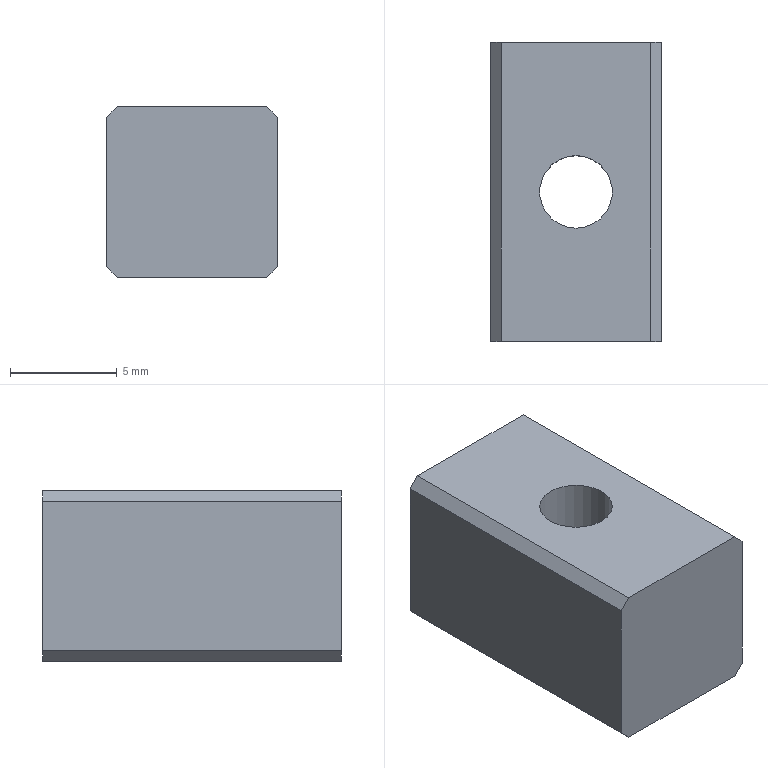Component | NX | LOCATING_KEY | 1 solid | 13 faces | box 8 x 14 x 8 mm | volume 732 mm3 | plane 11 | cylinder 2 | commonest cylinder face diameters 3.4 x1 6.5 x1
STEP:
#1=CARTESIAN_POINT('',(0.,0.,0.));
#2=DIRECTION('',(0.,0.,1.));
#3=DIRECTION('',(1.,0.,0.));
#4=AXIS2_PLACEMENT_3D('',#1,#2,#3);
#5=CARTESIAN_POINT('',(-3.5,90.,-0.));
#6=VERTEX_POINT('',#5);
#7=CARTESIAN_POINT('',(3.5,90.,-0.));
#8=VERTEX_POINT('',#7);
#9=CARTESIAN_POINT('',(-4.,90.,-0.));
#10=DIRECTION('',(1.,0.,0.));
#11=VECTOR('',#10,1.);
#12=LINE('',#9,#11);
#13=CARTESIAN_POINT('',(-4.,90.,-0.));
#14=DIRECTION('',(0.,1.,0.));
#15=DIRECTION('',(0.,0.,-1.));
#16=AXIS2_PLACEMENT_3D('',#13,#14,#15);
#17=PLANE('',#16);
#18=CARTESIAN_POINT('',(0.,0.));
#19=DIRECTION('',(0.,-1.));
#20=VECTOR('',#19,1.);
#21=LINE('',#18,#20);
#22=(GEOMETRIC_REPRESENTATION_CONTEXT(2)PARAMETRIC_REPRESENTATION_CONTEXT()REPRESENTATION_CONTEXT('',''));
#23=DEFINITIONAL_REPRESENTATION('',(#21),#22);
#24=PCURVE('',#17,#23);
#25=CARTESIAN_POINT('',(0.,97.,-0.));
#26=DIRECTION('',(0.,0.,1.));
#27=DIRECTION('',(0.,1.,0.));
#28=AXIS2_PLACEMENT_3D('',#25,#26,#27);
#29=PLANE('',#28);
#30=CARTESIAN_POINT('',(-7.,4.));
#31=DIRECTION('',(0.,-1.));
#32=VECTOR('',#31,1.);
#33=LINE('',#30,#32);
#34=(GEOMETRIC_REPRESENTATION_CONTEXT(2)PARAMETRIC_REPRESENTATION_CONTEXT()REPRESENTATION_CONTEXT('',''));
#35=DEFINITIONAL_REPRESENTATION('',(#33),#34);
#36=PCURVE('',#29,#35);
#37=SURFACE_CURVE('',#12,(#24,#36),.PCURVE_S1.);
#38=EDGE_CURVE('',#6,#8,#37,.T.);
#39=ORIENTED_EDGE('',*,*,#38,.F.);
#40=CARTESIAN_POINT('',(-4.,90.,-0.5));
#41=VERTEX_POINT('',#40);
#42=CARTESIAN_POINT('',(-3.5,90.,-0.));
#43=DIRECTION('',(-0.7071,0.,-0.7071));
#44=VECTOR('',#43,1.);
#45=LINE('',#42,#44);
#46=CARTESIAN_POINT('',(0.,-0.5));
#47=DIRECTION('',(0.7071,0.7071));
#48=VECTOR('',#47,1.);
#49=LINE('',#46,#48);
#50=(GEOMETRIC_REPRESENTATION_CONTEXT(2)PARAMETRIC_REPRESENTATION_CONTEXT()REPRESENTATION_CONTEXT('',''));
#51=DEFINITIONAL_REPRESENTATION('',(#49),#50);
#52=PCURVE('',#17,#51);
#53=CARTESIAN_POINT('',(-3.5,97.,-0.));
#54=DIRECTION('',(-0.7071,0.,0.7071));
#55=DIRECTION('',(0.,1.,0.));
#56=AXIS2_PLACEMENT_3D('',#53,#54,#55);
#57=PLANE('',#56);
#58=CARTESIAN_POINT('',(-7.,0.));
#59=DIRECTION('',(0.,1.));
#60=VECTOR('',#59,1.);
#61=LINE('',#58,#60);
#62=(GEOMETRIC_REPRESENTATION_CONTEXT(2)PARAMETRIC_REPRESENTATION_CONTEXT()REPRESENTATION_CONTEXT('',''));
#63=DEFINITIONAL_REPRESENTATION('',(#61),#62);
#64=PCURVE('',#57,#63);
#65=SURFACE_CURVE('',#45,(#52,#64),.PCURVE_S1.);
#66=EDGE_CURVE('',#6,#41,#65,.T.);
#67=ORIENTED_EDGE('',*,*,#66,.T.);
#68=CARTESIAN_POINT('',(-4.,90.,-7.5));
#69=VERTEX_POINT('',#68);
#70=CARTESIAN_POINT('',(-4.,90.,-0.));
#71=DIRECTION('',(0.,0.,-1.));
#72=VECTOR('',#71,1.);
#73=LINE('',#70,#72);
#74=CARTESIAN_POINT('',(0.,0.));
#75=DIRECTION('',(1.,0.));
#76=VECTOR('',#75,1.);
#77=LINE('',#74,#76);
#78=(GEOMETRIC_REPRESENTATION_CONTEXT(2)PARAMETRIC_REPRESENTATION_CONTEXT()REPRESENTATION_CONTEXT('',''));
#79=DEFINITIONAL_REPRESENTATION('',(#77),#78);
#80=PCURVE('',#17,#79);
#81=CARTESIAN_POINT('',(-4.,104.,-0.));
#82=DIRECTION('',(1.,0.,0.));
#83=DIRECTION('',(0.,0.,-1.));
#84=AXIS2_PLACEMENT_3D('',#81,#82,#83);
#85=PLANE('',#84);
#86=CARTESIAN_POINT('',(0.,-14.));
#87=DIRECTION('',(1.,0.));
#88=VECTOR('',#87,1.);
#89=LINE('',#86,#88);
#90=(GEOMETRIC_REPRESENTATION_CONTEXT(2)PARAMETRIC_REPRESENTATION_CONTEXT()REPRESENTATION_CONTEXT('',''));
#91=DEFINITIONAL_REPRESENTATION('',(#89),#90);
#92=PCURVE('',#85,#91);
#93=SURFACE_CURVE('',#73,(#80,#92),.PCURVE_S1.);
#94=EDGE_CURVE('',#41,#69,#93,.T.);
#95=ORIENTED_EDGE('',*,*,#94,.T.);
#96=CARTESIAN_POINT('',(-3.5,90.,-8.));
#97=VERTEX_POINT('',#96);
#98=CARTESIAN_POINT('',(-4.,90.,-7.5));
#99=DIRECTION('',(0.7071,0.,-0.7071));
#100=VECTOR('',#99,1.);
#101=LINE('',#98,#100);
#102=CARTESIAN_POINT('',(7.5,0.));
#103=DIRECTION('',(0.7071,-0.7071));
#104=VECTOR('',#103,1.);
#105=LINE('',#102,#104);
#106=(GEOMETRIC_REPRESENTATION_CONTEXT(2)PARAMETRIC_REPRESENTATION_CONTEXT()REPRESENTATION_CONTEXT('',''));
#107=DEFINITIONAL_REPRESENTATION('',(#105),#106);
#108=PCURVE('',#17,#107);
#109=CARTESIAN_POINT('',(-4.,104.,-7.5));
#110=DIRECTION('',(0.7071,0.,0.7071));
#111=DIRECTION('',(0.,-1.,0.));
#112=AXIS2_PLACEMENT_3D('',#109,#110,#111);
#113=PLANE('',#112);
#114=CARTESIAN_POINT('',(14.,0.));
#115=DIRECTION('',(0.,1.));
#116=VECTOR('',#115,1.);
#117=LINE('',#114,#116);
#118=(GEOMETRIC_REPRESENTATION_CONTEXT(2)PARAMETRIC_REPRESENTATION_CONTEXT()REPRESENTATION_CONTEXT('',''));
#119=DEFINITIONAL_REPRESENTATION('',(#117),#118);
#120=PCURVE('',#113,#119);
#121=SURFACE_CURVE('',#101,(#108,#120),.PCURVE_S1.);
#122=EDGE_CURVE('',#69,#97,#121,.T.);
#123=ORIENTED_EDGE('',*,*,#122,.T.);
#124=CARTESIAN_POINT('',(3.5,90.,-8.));
#125=VERTEX_POINT('',#124);
#126=CARTESIAN_POINT('',(-4.,90.,-8.));
#127=DIRECTION('',(1.,0.,0.));
#128=VECTOR('',#127,1.);
#129=LINE('',#126,#128);
#130=CARTESIAN_POINT('',(8.,0.));
#131=DIRECTION('',(0.,-1.));
#132=VECTOR('',#131,1.);
#133=LINE('',#130,#132);
#134=(GEOMETRIC_REPRESENTATION_CONTEXT(2)PARAMETRIC_REPRESENTATION_CONTEXT()REPRESENTATION_CONTEXT('',''));
#135=DEFINITIONAL_REPRESENTATION('',(#133),#134);
#136=PCURVE('',#17,#135);
#137=CARTESIAN_POINT('',(0.,97.,-8.));
#138=DIRECTION('',(0.,0.,1.));
#139=DIRECTION('',(0.,1.,0.));
#140=AXIS2_PLACEMENT_3D('',#137,#138,#139);
#141=PLANE('',#140);
#142=CARTESIAN_POINT('',(-7.,4.));
#143=DIRECTION('',(0.,-1.));
#144=VECTOR('',#143,1.);
#145=LINE('',#142,#144);
#146=(GEOMETRIC_REPRESENTATION_CONTEXT(2)PARAMETRIC_REPRESENTATION_CONTEXT()REPRESENTATION_CONTEXT('',''));
#147=DEFINITIONAL_REPRESENTATION('',(#145),#146);
#148=PCURVE('',#141,#147);
#149=SURFACE_CURVE('',#129,(#136,#148),.PCURVE_S1.);
#150=EDGE_CURVE('',#97,#125,#149,.T.);
#151=ORIENTED_EDGE('',*,*,#150,.T.);
#152=CARTESIAN_POINT('',(4.,90.,-7.5));
#153=VERTEX_POINT('',#152);
#154=CARTESIAN_POINT('',(4.,90.,-7.5));
#155=DIRECTION('',(0.7071,0.,0.7071));
#156=VECTOR('',#155,1.);
#157=LINE('',#154,#156);
#158=CARTESIAN_POINT('',(7.5,-8.));
#159=DIRECTION('',(-0.7071,-0.7071));
#160=VECTOR('',#159,1.);
#161=LINE('',#158,#160);
#162=(GEOMETRIC_REPRESENTATION_CONTEXT(2)PARAMETRIC_REPRESENTATION_CONTEXT()REPRESENTATION_CONTEXT('',''));
#163=DEFINITIONAL_REPRESENTATION('',(#161),#162);
#164=PCURVE('',#17,#163);
#165=CARTESIAN_POINT('',(4.,90.,-7.5));
#166=DIRECTION('',(-0.7071,0.,0.7071));
#167=DIRECTION('',(0.,1.,0.));
#168=AXIS2_PLACEMENT_3D('',#165,#166,#167);
#169=PLANE('',#168);
#170=CARTESIAN_POINT('',(0.,0.));
#171=DIRECTION('',(0.,-1.));
#172=VECTOR('',#171,1.);
#173=LINE('',#170,#172);
#174=(GEOMETRIC_REPRESENTATION_CONTEXT(2)PARAMETRIC_REPRESENTATION_CONTEXT()REPRESENTATION_CONTEXT('',''));
#175=DEFINITIONAL_REPRESENTATION('',(#173),#174);
#176=PCURVE('',#169,#175);
#177=SURFACE_CURVE('',#157,(#164,#176),.PCURVE_S1.);
#178=EDGE_CURVE('',#125,#153,#177,.T.);
#179=ORIENTED_EDGE('',*,*,#178,.T.);
#180=CARTESIAN_POINT('',(4.,90.,-0.5));
#181=VERTEX_POINT('',#180);
#182=CARTESIAN_POINT('',(4.,90.,-0.));
#183=DIRECTION('',(0.,0.,-1.));
#184=VECTOR('',#183,1.);
#185=LINE('',#182,#184);
#186=CARTESIAN_POINT('',(0.,-8.));
#187=DIRECTION('',(1.,0.));
#188=VECTOR('',#187,1.);
#189=LINE('',#186,#188);
#190=(GEOMETRIC_REPRESENTATION_CONTEXT(2)PARAMETRIC_REPRESENTATION_CONTEXT()REPRESENTATION_CONTEXT('',''));
#191=DEFINITIONAL_REPRESENTATION('',(#189),#190);
#192=PCURVE('',#17,#191);
#193=CARTESIAN_POINT('',(4.,90.,-0.));
#194=DIRECTION('',(-1.,0.,0.));
#195=DIRECTION('',(0.,0.,1.));
#196=AXIS2_PLACEMENT_3D('',#193,#194,#195);
#197=PLANE('',#196);
#198=CARTESIAN_POINT('',(0.,0.));
#199=DIRECTION('',(-1.,0.));
#200=VECTOR('',#199,1.);
#201=LINE('',#198,#200);
#202=(GEOMETRIC_REPRESENTATION_CONTEXT(2)PARAMETRIC_REPRESENTATION_CONTEXT()REPRESENTATION_CONTEXT('',''));
#203=DEFINITIONAL_REPRESENTATION('',(#201),#202);
#204=PCURVE('',#197,#203);
#205=SURFACE_CURVE('',#185,(#192,#204),.PCURVE_S1.);
#206=EDGE_CURVE('',#181,#153,#205,.T.);
#207=ORIENTED_EDGE('',*,*,#206,.F.);
#208=CARTESIAN_POINT('',(3.5,90.,-0.));
#209=DIRECTION('',(-0.7071,0.,0.7071));
#210=VECTOR('',#209,1.);
#211=LINE('',#208,#210);
#212=CARTESIAN_POINT('',(0.,-7.5));
#213=DIRECTION('',(-0.7071,0.7071));
#214=VECTOR('',#213,1.);
#215=LINE('',#212,#214);
#216=(GEOMETRIC_REPRESENTATION_CONTEXT(2)PARAMETRIC_REPRESENTATION_CONTEXT()REPRESENTATION_CONTEXT('',''));
#217=DEFINITIONAL_REPRESENTATION('',(#215),#216);
#218=PCURVE('',#17,#217);
#219=CARTESIAN_POINT('',(3.5,97.,-0.));
#220=DIRECTION('',(0.7071,0.,0.7071));
#221=DIRECTION('',(0.,-1.,0.));
#222=AXIS2_PLACEMENT_3D('',#219,#220,#221);
#223=PLANE('',#222);
#224=CARTESIAN_POINT('',(7.,0.));
#225=DIRECTION('',(0.,-1.));
#226=VECTOR('',#225,1.);
#227=LINE('',#224,#226);
#228=(GEOMETRIC_REPRESENTATION_CONTEXT(2)PARAMETRIC_REPRESENTATION_CONTEXT()REPRESENTATION_CONTEXT('',''));
#229=DEFINITIONAL_REPRESENTATION('',(#227),#228);
#230=PCURVE('',#223,#229);
#231=SURFACE_CURVE('',#211,(#218,#230),.PCURVE_S1.);
#232=EDGE_CURVE('',#181,#8,#231,.T.);
#233=ORIENTED_EDGE('',*,*,#232,.T.);
#234=EDGE_LOOP('',(#39,#67,#95,#123,#151,#179,#207,#233));
#235=FACE_BOUND('',#234,.T.);
#236=ADVANCED_FACE('',(#235),#17,.F.);
#237=ORIENTED_EDGE('',*,*,#206,.T.);
#238=CARTESIAN_POINT('',(4.,104.,-7.5));
#239=VERTEX_POINT('',#238);
#240=CARTESIAN_POINT('',(4.,90.,-7.5));
#241=DIRECTION('',(0.,1.,0.));
#242=VECTOR('',#241,1.);
#243=LINE('',#240,#242);
#244=CARTESIAN_POINT('',(-7.5,0.));
#245=DIRECTION('',(0.,1.));
#246=VECTOR('',#245,1.);
#247=LINE('',#244,#246);
#248=(GEOMETRIC_REPRESENTATION_CONTEXT(2)PARAMETRIC_REPRESENTATION_CONTEXT()REPRESENTATION_CONTEXT('',''));
#249=DEFINITIONAL_REPRESENTATION('',(#247),#248);
#250=PCURVE('',#197,#249);
#251=CARTESIAN_POINT('',(0.,0.));
#252=DIRECTION('',(1.,0.));
#253=VECTOR('',#252,1.);
#254=LINE('',#251,#253);
#255=(GEOMETRIC_REPRESENTATION_CONTEXT(2)PARAMETRIC_REPRESENTATION_CONTEXT()REPRESENTATION_CONTEXT('',''));
#256=DEFINITIONAL_REPRESENTATION('',(#254),#255);
#257=PCURVE('',#169,#256);
#258=SURFACE_CURVE('',#243,(#250,#257),.PCURVE_S1.);
#259=EDGE_CURVE('',#153,#239,#258,.T.);
#260=ORIENTED_EDGE('',*,*,#259,.T.);
#261=CARTESIAN_POINT('',(4.,104.,-0.5));
#262=VERTEX_POINT('',#261);
#263=CARTESIAN_POINT('',(4.,104.,-0.));
#264=DIRECTION('',(0.,0.,-1.));
#265=VECTOR('',#264,1.);
#266=LINE('',#263,#265);
#267=CARTESIAN_POINT('',(0.,14.));
#268=DIRECTION('',(-1.,0.));
#269=VECTOR('',#268,1.);
#270=LINE('',#267,#269);
#271=(GEOMETRIC_REPRESENTATION_CONTEXT(2)PARAMETRIC_REPRESENTATION_CONTEXT()REPRESENTATION_CONTEXT('',''));
#272=DEFINITIONAL_REPRESENTATION('',(#270),#271);
#273=PCURVE('',#197,#272);
#274=CARTESIAN_POINT('',(4.,104.,-0.));
#275=DIRECTION('',(0.,-1.,0.));
#276=DIRECTION('',(0.,0.,1.));
#277=AXIS2_PLACEMENT_3D('',#274,#275,#276);
#278=PLANE('',#277);
#279=CARTESIAN_POINT('',(0.,0.));
#280=DIRECTION('',(-1.,0.));
#281=VECTOR('',#280,1.);
#282=LINE('',#279,#281);
#283=(GEOMETRIC_REPRESENTATION_CONTEXT(2)PARAMETRIC_REPRESENTATION_CONTEXT()REPRESENTATION_CONTEXT('',''));
#284=DEFINITIONAL_REPRESENTATION('',(#282),#283);
#285=PCURVE('',#278,#284);
#286=SURFACE_CURVE('',#266,(#273,#285),.PCURVE_S1.);
#287=EDGE_CURVE('',#262,#239,#286,.T.);
#288=ORIENTED_EDGE('',*,*,#287,.F.);
#289=CARTESIAN_POINT('',(4.,90.,-0.5));
#290=DIRECTION('',(0.,-1.,0.));
#291=VECTOR('',#290,1.);
#292=LINE('',#289,#291);
#293=CARTESIAN_POINT('',(-0.5,0.));
#294=DIRECTION('',(0.,-1.));
#295=VECTOR('',#294,1.);
#296=LINE('',#293,#295);
#297=(GEOMETRIC_REPRESENTATION_CONTEXT(2)PARAMETRIC_REPRESENTATION_CONTEXT()REPRESENTATION_CONTEXT('',''));
#298=DEFINITIONAL_REPRESENTATION('',(#296),#297);
#299=PCURVE('',#197,#298);
#300=CARTESIAN_POINT('',(7.,0.7071));
#301=DIRECTION('',(1.,0.));
#302=VECTOR('',#301,1.);
#303=LINE('',#300,#302);
#304=(GEOMETRIC_REPRESENTATION_CONTEXT(2)PARAMETRIC_REPRESENTATION_CONTEXT()REPRESENTATION_CONTEXT('',''));
#305=DEFINITIONAL_REPRESENTATION('',(#303),#304);
#306=PCURVE('',#223,#305);
#307=SURFACE_CURVE('',#292,(#299,#306),.PCURVE_S1.);
#308=EDGE_CURVE('',#262,#181,#307,.T.);
#309=ORIENTED_EDGE('',*,*,#308,.T.);
#310=EDGE_LOOP('',(#237,#260,#288,#309));
#311=FACE_BOUND('',#310,.T.);
#312=ADVANCED_FACE('',(#311),#197,.F.);
#313=CARTESIAN_POINT('',(-4.,104.,-0.5));
#314=VERTEX_POINT('',#313);
#315=CARTESIAN_POINT('',(-4.,104.,-7.5));
#316=VERTEX_POINT('',#315);
#317=CARTESIAN_POINT('',(-4.,104.,-0.));
#318=DIRECTION('',(0.,0.,-1.));
#319=VECTOR('',#318,1.);
#320=LINE('',#317,#319);
#321=CARTESIAN_POINT('',(0.,8.));
#322=DIRECTION('',(-1.,0.));
#323=VECTOR('',#322,1.);
#324=LINE('',#321,#323);
#325=(GEOMETRIC_REPRESENTATION_CONTEXT(2)PARAMETRIC_REPRESENTATION_CONTEXT()REPRESENTATION_CONTEXT('',''));
#326=DEFINITIONAL_REPRESENTATION('',(#324),#325);
#327=PCURVE('',#278,#326);
#328=CARTESIAN_POINT('',(0.,0.));
#329=DIRECTION('',(1.,0.));
#330=VECTOR('',#329,1.);
#331=LINE('',#328,#330);
#332=(GEOMETRIC_REPRESENTATION_CONTEXT(2)PARAMETRIC_REPRESENTATION_CONTEXT()REPRESENTATION_CONTEXT('',''));
#333=DEFINITIONAL_REPRESENTATION('',(#331),#332);
#334=PCURVE('',#85,#333);
#335=SURFACE_CURVE('',#320,(#327,#334),.PCURVE_S1.);
#336=EDGE_CURVE('',#314,#316,#335,.T.);
#337=ORIENTED_EDGE('',*,*,#336,.F.);
#338=CARTESIAN_POINT('',(-3.5,104.,-0.));
#339=VERTEX_POINT('',#338);
#340=CARTESIAN_POINT('',(-3.5,104.,-0.));
#341=DIRECTION('',(0.7071,0.,0.7071));
#342=VECTOR('',#341,1.);
#343=LINE('',#340,#342);
#344=CARTESIAN_POINT('',(0.,7.5));
#345=DIRECTION('',(0.7071,-0.7071));
#346=VECTOR('',#345,1.);
#347=LINE('',#344,#346);
#348=(GEOMETRIC_REPRESENTATION_CONTEXT(2)PARAMETRIC_REPRESENTATION_CONTEXT()REPRESENTATION_CONTEXT('',''));
#349=DEFINITIONAL_REPRESENTATION('',(#347),#348);
#350=PCURVE('',#278,#349);
#351=CARTESIAN_POINT('',(7.,0.));
#352=DIRECTION('',(0.,-1.));
#353=VECTOR('',#352,1.);
#354=LINE('',#351,#353);
#355=(GEOMETRIC_REPRESENTATION_CONTEXT(2)PARAMETRIC_REPRESENTATION_CONTEXT()REPRESENTATION_CONTEXT('',''));
#356=DEFINITIONAL_REPRESENTATION('',(#354),#355);
#357=PCURVE('',#57,#356);
#358=SURFACE_CURVE('',#343,(#350,#357),.PCURVE_S1.);
#359=EDGE_CURVE('',#314,#339,#358,.T.);
#360=ORIENTED_EDGE('',*,*,#359,.T.);
#361=CARTESIAN_POINT('',(3.5,104.,-0.));
#362=VERTEX_POINT('',#361);
#363=CARTESIAN_POINT('',(4.,104.,-0.));
#364=DIRECTION('',(-1.,0.,0.));
#365=VECTOR('',#364,1.);
#366=LINE('',#363,#365);
#367=CARTESIAN_POINT('',(0.,0.));
#368=DIRECTION('',(0.,1.));
#369=VECTOR('',#368,1.);
#370=LINE('',#367,#369);
#371=(GEOMETRIC_REPRESENTATION_CONTEXT(2)PARAMETRIC_REPRESENTATION_CONTEXT()REPRESENTATION_CONTEXT('',''));
#372=DEFINITIONAL_REPRESENTATION('',(#370),#371);
#373=PCURVE('',#278,#372);
#374=CARTESIAN_POINT('',(7.,-4.));
#375=DIRECTION('',(0.,1.));
#376=VECTOR('',#375,1.);
#377=LINE('',#374,#376);
#378=(GEOMETRIC_REPRESENTATION_CONTEXT(2)PARAMETRIC_REPRESENTATION_CONTEXT()REPRESENTATION_CONTEXT('',''));
#379=DEFINITIONAL_REPRESENTATION('',(#377),#378);
#380=PCURVE('',#29,#379);
#381=SURFACE_CURVE('',#366,(#373,#380),.PCURVE_S1.);
#382=EDGE_CURVE('',#362,#339,#381,.T.);
#383=ORIENTED_EDGE('',*,*,#382,.F.);
#384=CARTESIAN_POINT('',(3.5,104.,-0.));
#385=DIRECTION('',(0.7071,0.,-0.7071));
#386=VECTOR('',#385,1.);
#387=LINE('',#384,#386);
#388=CARTESIAN_POINT('',(0.,0.5));
#389=DIRECTION('',(-0.7071,-0.7071));
#390=VECTOR('',#389,1.);
#391=LINE('',#388,#390);
#392=(GEOMETRIC_REPRESENTATION_CONTEXT(2)PARAMETRIC_REPRESENTATION_CONTEXT()REPRESENTATION_CONTEXT('',''));
#393=DEFINITIONAL_REPRESENTATION('',(#391),#392);
#394=PCURVE('',#278,#393);
#395=CARTESIAN_POINT('',(-7.,0.));
#396=DIRECTION('',(0.,1.));
#397=VECTOR('',#396,1.);
#398=LINE('',#395,#397);
#399=(GEOMETRIC_REPRESENTATION_CONTEXT(2)PARAMETRIC_REPRESENTATION_CONTEXT()REPRESENTATION_CONTEXT('',''));
#400=DEFINITIONAL_REPRESENTATION('',(#398),#399);
#401=PCURVE('',#223,#400);
#402=SURFACE_CURVE('',#387,(#394,#401),.PCURVE_S1.);
#403=EDGE_CURVE('',#362,#262,#402,.T.);
#404=ORIENTED_EDGE('',*,*,#403,.T.);
#405=ORIENTED_EDGE('',*,*,#287,.T.);
#406=CARTESIAN_POINT('',(3.5,104.,-8.));
#407=VERTEX_POINT('',#406);
#408=CARTESIAN_POINT('',(4.,104.,-7.5));
#409=DIRECTION('',(-0.7071,0.,-0.7071));
#410=VECTOR('',#409,1.);
#411=LINE('',#408,#410);
#412=CARTESIAN_POINT('',(-7.5,0.));
#413=DIRECTION('',(-0.7071,0.7071));
#414=VECTOR('',#413,1.);
#415=LINE('',#412,#414);
#416=(GEOMETRIC_REPRESENTATION_CONTEXT(2)PARAMETRIC_REPRESENTATION_CONTEXT()REPRESENTATION_CONTEXT('',''));
#417=DEFINITIONAL_REPRESENTATION('',(#415),#416);
#418=PCURVE('',#278,#417);
#419=CARTESIAN_POINT('',(14.,0.));
#420=DIRECTION('',(0.,1.));
#421=VECTOR('',#420,1.);
#422=LINE('',#419,#421);
#423=(GEOMETRIC_REPRESENTATION_CONTEXT(2)PARAMETRIC_REPRESENTATION_CONTEXT()REPRESENTATION_CONTEXT('',''));
#424=DEFINITIONAL_REPRESENTATION('',(#422),#423);
#425=PCURVE('',#169,#424);
#426=SURFACE_CURVE('',#411,(#418,#425),.PCURVE_S1.);
#427=EDGE_CURVE('',#239,#407,#426,.T.);
#428=ORIENTED_EDGE('',*,*,#427,.T.);
#429=CARTESIAN_POINT('',(-3.5,104.,-8.));
#430=VERTEX_POINT('',#429);
#431=CARTESIAN_POINT('',(4.,104.,-8.));
#432=DIRECTION('',(-1.,0.,0.));
#433=VECTOR('',#432,1.);
#434=LINE('',#431,#433);
#435=CARTESIAN_POINT('',(-8.,0.));
#436=DIRECTION('',(0.,1.));
#437=VECTOR('',#436,1.);
#438=LINE('',#435,#437);
#439=(GEOMETRIC_REPRESENTATION_CONTEXT(2)PARAMETRIC_REPRESENTATION_CONTEXT()REPRESENTATION_CONTEXT('',''));
#440=DEFINITIONAL_REPRESENTATION('',(#438),#439);
#441=PCURVE('',#278,#440);
#442=CARTESIAN_POINT('',(7.,-4.));
#443=DIRECTION('',(0.,1.));
#444=VECTOR('',#443,1.);
#445=LINE('',#442,#444);
#446=(GEOMETRIC_REPRESENTATION_CONTEXT(2)PARAMETRIC_REPRESENTATION_CONTEXT()REPRESENTATION_CONTEXT('',''));
#447=DEFINITIONAL_REPRESENTATION('',(#445),#446);
#448=PCURVE('',#141,#447);
#449=SURFACE_CURVE('',#434,(#441,#448),.PCURVE_S1.);
#450=EDGE_CURVE('',#407,#430,#449,.T.);
#451=ORIENTED_EDGE('',*,*,#450,.T.);
#452=CARTESIAN_POINT('',(-4.,104.,-7.5));
#453=DIRECTION('',(-0.7071,0.,0.7071));
#454=VECTOR('',#453,1.);
#455=LINE('',#452,#454);
#456=CARTESIAN_POINT('',(-7.5,8.));
#457=DIRECTION('',(0.7071,0.7071));
#458=VECTOR('',#457,1.);
#459=LINE('',#456,#458);
#460=(GEOMETRIC_REPRESENTATION_CONTEXT(2)PARAMETRIC_REPRESENTATION_CONTEXT()REPRESENTATION_CONTEXT('',''));
#461=DEFINITIONAL_REPRESENTATION('',(#459),#460);
#462=PCURVE('',#278,#461);
#463=CARTESIAN_POINT('',(0.,0.));
#464=DIRECTION('',(0.,-1.));
#465=VECTOR('',#464,1.);
#466=LINE('',#463,#465);
#467=(GEOMETRIC_REPRESENTATION_CONTEXT(2)PARAMETRIC_REPRESENTATION_CONTEXT()REPRESENTATION_CONTEXT('',''));
#468=DEFINITIONAL_REPRESENTATION('',(#466),#467);
#469=PCURVE('',#113,#468);
#470=SURFACE_CURVE('',#455,(#462,#469),.PCURVE_S1.);
#471=EDGE_CURVE('',#430,#316,#470,.T.);
#472=ORIENTED_EDGE('',*,*,#471,.T.);
#473=EDGE_LOOP('',(#337,#360,#383,#404,#405,#428,#451,#472));
#474=FACE_BOUND('',#473,.T.);
#475=ADVANCED_FACE('',(#474),#278,.F.);
#476=ORIENTED_EDGE('',*,*,#94,.F.);
#477=CARTESIAN_POINT('',(-4.,104.,-0.5));
#478=DIRECTION('',(0.,1.,0.));
#479=VECTOR('',#478,1.);
#480=LINE('',#477,#479);
#481=CARTESIAN_POINT('',(0.5,0.));
#482=DIRECTION('',(0.,1.));
#483=VECTOR('',#482,1.);
#484=LINE('',#481,#483);
#485=(GEOMETRIC_REPRESENTATION_CONTEXT(2)PARAMETRIC_REPRESENTATION_CONTEXT()REPRESENTATION_CONTEXT('',''));
#486=DEFINITIONAL_REPRESENTATION('',(#484),#485);
#487=PCURVE('',#85,#486);
#488=CARTESIAN_POINT('',(7.,0.7071));
#489=DIRECTION('',(1.,0.));
#490=VECTOR('',#489,1.);
#491=LINE('',#488,#490);
#492=(GEOMETRIC_REPRESENTATION_CONTEXT(2)PARAMETRIC_REPRESENTATION_CONTEXT()REPRESENTATION_CONTEXT('',''));
#493=DEFINITIONAL_REPRESENTATION('',(#491),#492);
#494=PCURVE('',#57,#493);
#495=SURFACE_CURVE('',#480,(#487,#494),.PCURVE_S1.);
#496=EDGE_CURVE('',#41,#314,#495,.T.);
#497=ORIENTED_EDGE('',*,*,#496,.T.);
#498=ORIENTED_EDGE('',*,*,#336,.T.);
#499=CARTESIAN_POINT('',(-4.,104.,-7.5));
#500=DIRECTION('',(0.,-1.,0.));
#501=VECTOR('',#500,1.);
#502=LINE('',#499,#501);
#503=CARTESIAN_POINT('',(7.5,0.));
#504=DIRECTION('',(0.,-1.));
#505=VECTOR('',#504,1.);
#506=LINE('',#503,#505);
#507=(GEOMETRIC_REPRESENTATION_CONTEXT(2)PARAMETRIC_REPRESENTATION_CONTEXT()REPRESENTATION_CONTEXT('',''));
#508=DEFINITIONAL_REPRESENTATION('',(#506),#507);
#509=PCURVE('',#85,#508);
#510=CARTESIAN_POINT('',(0.,0.));
#511=DIRECTION('',(1.,0.));
#512=VECTOR('',#511,1.);
#513=LINE('',#510,#512);
#514=(GEOMETRIC_REPRESENTATION_CONTEXT(2)PARAMETRIC_REPRESENTATION_CONTEXT()REPRESENTATION_CONTEXT('',''));
#515=DEFINITIONAL_REPRESENTATION('',(#513),#514);
#516=PCURVE('',#113,#515);
#517=SURFACE_CURVE('',#502,(#509,#516),.PCURVE_S1.);
#518=EDGE_CURVE('',#316,#69,#517,.T.);
#519=ORIENTED_EDGE('',*,*,#518,.T.);
#520=EDGE_LOOP('',(#476,#497,#498,#519));
#521=FACE_BOUND('',#520,.T.);
#522=ADVANCED_FACE('',(#521),#85,.F.);
#523=CARTESIAN_POINT('',(0.,98.7,-0.));
#524=VERTEX_POINT('',#523);
#525=CARTESIAN_POINT('',(0.,97.,-0.));
#526=DIRECTION('',(0.,0.,1.));
#527=DIRECTION('',(0.,1.,0.));
#528=AXIS2_PLACEMENT_3D('',#525,#526,#527);
#529=CIRCLE('',#528,1.7);
#530=CARTESIAN_POINT('',(0.,0.));
#531=DIRECTION('',(1.,0.));
#532=AXIS2_PLACEMENT_2D('',#530,#531);
#533=CIRCLE('',#532,1.7);
#534=(GEOMETRIC_REPRESENTATION_CONTEXT(2)PARAMETRIC_REPRESENTATION_CONTEXT()REPRESENTATION_CONTEXT('',''));
#535=DEFINITIONAL_REPRESENTATION('',(#533),#534);
#536=PCURVE('',#29,#535);
#537=CARTESIAN_POINT('',(0.,97.,5.9));
#538=DIRECTION('',(0.,0.,1.));
#539=DIRECTION('',(0.,1.,0.));
#540=AXIS2_PLACEMENT_3D('',#537,#538,#539);
#541=CYLINDRICAL_SURFACE('',#540,1.7);
#542=CARTESIAN_POINT('',(0.,-5.9));
#543=DIRECTION('',(1.,0.));
#544=VECTOR('',#543,1.);
#545=LINE('',#542,#544);
#546=(GEOMETRIC_REPRESENTATION_CONTEXT(2)PARAMETRIC_REPRESENTATION_CONTEXT()REPRESENTATION_CONTEXT('',''));
#547=DEFINITIONAL_REPRESENTATION('',(#545),#546);
#548=PCURVE('',#541,#547);
#549=SURFACE_CURVE('',#529,(#536,#548),.PCURVE_S1.);
#550=EDGE_CURVE('',#524,#524,#549,.T.);
#551=ORIENTED_EDGE('',*,*,#550,.F.);
#552=EDGE_LOOP('',(#551));
#553=FACE_BOUND('',#552,.T.);
#554=ORIENTED_EDGE('',*,*,#382,.T.);
#555=CARTESIAN_POINT('',(-3.5,90.,-0.));
#556=DIRECTION('',(0.,-1.,0.));
#557=VECTOR('',#556,1.);
#558=LINE('',#555,#557);
#559=CARTESIAN_POINT('',(-7.,3.5));
#560=DIRECTION('',(-1.,0.));
#561=VECTOR('',#560,1.);
#562=LINE('',#559,#561);
#563=(GEOMETRIC_REPRESENTATION_CONTEXT(2)PARAMETRIC_REPRESENTATION_CONTEXT()REPRESENTATION_CONTEXT('',''));
#564=DEFINITIONAL_REPRESENTATION('',(#562),#563);
#565=PCURVE('',#29,#564);
#566=CARTESIAN_POINT('',(-7.,0.));
#567=DIRECTION('',(-1.,0.));
#568=VECTOR('',#567,1.);
#569=LINE('',#566,#568);
#570=(GEOMETRIC_REPRESENTATION_CONTEXT(2)PARAMETRIC_REPRESENTATION_CONTEXT()REPRESENTATION_CONTEXT('',''));
#571=DEFINITIONAL_REPRESENTATION('',(#569),#570);
#572=PCURVE('',#57,#571);
#573=SURFACE_CURVE('',#558,(#565,#572),.PCURVE_S1.);
#574=EDGE_CURVE('',#339,#6,#573,.T.);
#575=ORIENTED_EDGE('',*,*,#574,.T.);
#576=ORIENTED_EDGE('',*,*,#38,.T.);
#577=CARTESIAN_POINT('',(3.5,104.,-0.));
#578=DIRECTION('',(0.,1.,0.));
#579=VECTOR('',#578,1.);
#580=LINE('',#577,#579);
#581=CARTESIAN_POINT('',(7.,-3.5));
#582=DIRECTION('',(1.,0.));
#583=VECTOR('',#582,1.);
#584=LINE('',#581,#583);
#585=(GEOMETRIC_REPRESENTATION_CONTEXT(2)PARAMETRIC_REPRESENTATION_CONTEXT()REPRESENTATION_CONTEXT('',''));
#586=DEFINITIONAL_REPRESENTATION('',(#584),#585);
#587=PCURVE('',#29,#586);
#588=CARTESIAN_POINT('',(-7.,0.));
#589=DIRECTION('',(-1.,0.));
#590=VECTOR('',#589,1.);
#591=LINE('',#588,#590);
#592=(GEOMETRIC_REPRESENTATION_CONTEXT(2)PARAMETRIC_REPRESENTATION_CONTEXT()REPRESENTATION_CONTEXT('',''));
#593=DEFINITIONAL_REPRESENTATION('',(#591),#592);
#594=PCURVE('',#223,#593);
#595=SURFACE_CURVE('',#580,(#587,#594),.PCURVE_S1.);
#596=EDGE_CURVE('',#8,#362,#595,.T.);
#597=ORIENTED_EDGE('',*,*,#596,.T.);
#598=EDGE_LOOP('',(#554,#575,#576,#597));
#599=FACE_BOUND('',#598,.T.);
#600=ADVANCED_FACE('',(#553,#599),#29,.T.);
#601=CARTESIAN_POINT('',(0.,100.25,-8.));
#602=VERTEX_POINT('',#601);
#603=CARTESIAN_POINT('',(0.,97.,-8.));
#604=DIRECTION('',(0.,0.,1.));
#605=DIRECTION('',(0.,1.,0.));
#606=AXIS2_PLACEMENT_3D('',#603,#604,#605);
#607=CIRCLE('',#606,3.25);
#608=CARTESIAN_POINT('',(0.,0.));
#609=DIRECTION('',(1.,0.));
#610=AXIS2_PLACEMENT_2D('',#608,#609);
#611=CIRCLE('',#610,3.25);
#612=(GEOMETRIC_REPRESENTATION_CONTEXT(2)PARAMETRIC_REPRESENTATION_CONTEXT()REPRESENTATION_CONTEXT('',''));
#613=DEFINITIONAL_REPRESENTATION('',(#611),#612);
#614=PCURVE('',#141,#613);
#615=CARTESIAN_POINT('',(0.,97.,-8.));
#616=DIRECTION('',(0.,0.,1.));
#617=DIRECTION('',(0.,1.,0.));
#618=AXIS2_PLACEMENT_3D('',#615,#616,#617);
#619=CYLINDRICAL_SURFACE('',#618,3.25);
#620=CARTESIAN_POINT('',(0.,0.));
#621=DIRECTION('',(1.,0.));
#622=VECTOR('',#621,1.);
#623=LINE('',#620,#622);
#624=(GEOMETRIC_REPRESENTATION_CONTEXT(2)PARAMETRIC_REPRESENTATION_CONTEXT()REPRESENTATION_CONTEXT('',''));
#625=DEFINITIONAL_REPRESENTATION('',(#623),#624);
#626=PCURVE('',#619,#625);
#627=SURFACE_CURVE('',#607,(#614,#626),.PCURVE_S1.);
#628=EDGE_CURVE('',#602,#602,#627,.T.);
#629=ORIENTED_EDGE('',*,*,#628,.T.);
#630=EDGE_LOOP('',(#629));
#631=FACE_BOUND('',#630,.T.);
#632=ORIENTED_EDGE('',*,*,#150,.F.);
#633=CARTESIAN_POINT('',(-3.5,97.,-8.));
#634=DIRECTION('',(0.,1.,0.));
#635=VECTOR('',#634,1.);
#636=LINE('',#633,#635);
#637=CARTESIAN_POINT('',(0.,3.5));
#638=DIRECTION('',(1.,0.));
#639=VECTOR('',#638,1.);
#640=LINE('',#637,#639);
#641=(GEOMETRIC_REPRESENTATION_CONTEXT(2)PARAMETRIC_REPRESENTATION_CONTEXT()REPRESENTATION_CONTEXT('',''));
#642=DEFINITIONAL_REPRESENTATION('',(#640),#641);
#643=PCURVE('',#141,#642);
#644=CARTESIAN_POINT('',(7.,0.7071));
#645=DIRECTION('',(-1.,0.));
#646=VECTOR('',#645,1.);
#647=LINE('',#644,#646);
#648=(GEOMETRIC_REPRESENTATION_CONTEXT(2)PARAMETRIC_REPRESENTATION_CONTEXT()REPRESENTATION_CONTEXT('',''));
#649=DEFINITIONAL_REPRESENTATION('',(#647),#648);
#650=PCURVE('',#113,#649);
#651=SURFACE_CURVE('',#636,(#643,#650),.PCURVE_S1.);
#652=EDGE_CURVE('',#97,#430,#651,.T.);
#653=ORIENTED_EDGE('',*,*,#652,.T.);
#654=ORIENTED_EDGE('',*,*,#450,.F.);
#655=CARTESIAN_POINT('',(3.5,97.,-8.));
#656=DIRECTION('',(0.,-1.,0.));
#657=VECTOR('',#656,1.);
#658=LINE('',#655,#657);
#659=CARTESIAN_POINT('',(0.,-3.5));
#660=DIRECTION('',(-1.,0.));
#661=VECTOR('',#660,1.);
#662=LINE('',#659,#661);
#663=(GEOMETRIC_REPRESENTATION_CONTEXT(2)PARAMETRIC_REPRESENTATION_CONTEXT()REPRESENTATION_CONTEXT('',''));
#664=DEFINITIONAL_REPRESENTATION('',(#662),#663);
#665=PCURVE('',#141,#664);
#666=CARTESIAN_POINT('',(7.,0.7071));
#667=DIRECTION('',(-1.,0.));
#668=VECTOR('',#667,1.);
#669=LINE('',#666,#668);
#670=(GEOMETRIC_REPRESENTATION_CONTEXT(2)PARAMETRIC_REPRESENTATION_CONTEXT()REPRESENTATION_CONTEXT('',''));
#671=DEFINITIONAL_REPRESENTATION('',(#669),#670);
#672=PCURVE('',#169,#671);
#673=SURFACE_CURVE('',#658,(#665,#672),.PCURVE_S1.);
#674=EDGE_CURVE('',#407,#125,#673,.T.);
#675=ORIENTED_EDGE('',*,*,#674,.T.);
#676=EDGE_LOOP('',(#632,#653,#654,#675));
#677=FACE_BOUND('',#676,.T.);
#678=ADVANCED_FACE('',(#631,#677),#141,.F.);
#679=ORIENTED_EDGE('',*,*,#550,.F.);
#680=CARTESIAN_POINT('',(0.,98.7,-4.5));
#681=VERTEX_POINT('',#680);
#682=CARTESIAN_POINT('',(0.,98.7,-4.5));
#683=CARTESIAN_POINT('',(0.,98.7,-0.));
#684=B_SPLINE_CURVE_WITH_KNOTS('',1,(#682,#683),.UNSPECIFIED.,.F.,.F.,(2,2),(-10.4,-5.9),.PIECEWISE_BEZIER_KNOTS.);
#685=CARTESIAN_POINT('',(0.,0.));
#686=DIRECTION('',(0.,1.));
#687=VECTOR('',#686,1.);
#688=LINE('',#685,#687);
#689=(GEOMETRIC_REPRESENTATION_CONTEXT(2)PARAMETRIC_REPRESENTATION_CONTEXT()REPRESENTATION_CONTEXT('',''));
#690=DEFINITIONAL_REPRESENTATION('',(#688),#689);
#691=PCURVE('',#541,#690);
#692=CARTESIAN_POINT('',(6.283,0.));
#693=DIRECTION('',(0.,1.));
#694=VECTOR('',#693,1.);
#695=LINE('',#692,#694);
#696=(GEOMETRIC_REPRESENTATION_CONTEXT(2)PARAMETRIC_REPRESENTATION_CONTEXT()REPRESENTATION_CONTEXT('',''));
#697=DEFINITIONAL_REPRESENTATION('',(#695),#696);
#698=PCURVE('',#541,#697);
#699=SEAM_CURVE('',#684,(#691,#698),.PCURVE_S1.);
#700=EDGE_CURVE('',#681,#524,#699,.T.);
#701=ORIENTED_EDGE('',*,*,#700,.F.);
#702=CARTESIAN_POINT('',(0.,97.,-4.5));
#703=DIRECTION('',(0.,0.,-1.));
#704=DIRECTION('',(0.,1.,0.));
#705=AXIS2_PLACEMENT_3D('',#702,#703,#704);
#706=CIRCLE('',#705,1.7);
#707=CARTESIAN_POINT('',(6.283,-10.4));
#708=DIRECTION('',(-1.,0.));
#709=VECTOR('',#708,1.);
#710=LINE('',#707,#709);
#711=(GEOMETRIC_REPRESENTATION_CONTEXT(2)PARAMETRIC_REPRESENTATION_CONTEXT()REPRESENTATION_CONTEXT('',''));
#712=DEFINITIONAL_REPRESENTATION('',(#710),#711);
#713=PCURVE('',#541,#712);
#714=CARTESIAN_POINT('',(0.,97.,-4.5));
#715=DIRECTION('',(0.,0.,1.));
#716=DIRECTION('',(0.,1.,0.));
#717=AXIS2_PLACEMENT_3D('',#714,#715,#716);
#718=PLANE('',#717);
#719=CARTESIAN_POINT('',(1.7,0.));
#720=CARTESIAN_POINT('',(1.7,-2.944));
#721=CARTESIAN_POINT('',(-0.85,-1.472));
#722=CARTESIAN_POINT('',(-3.4,-0.));
#723=CARTESIAN_POINT('',(-0.85,1.472));
#724=CARTESIAN_POINT('',(1.7,2.944));
#725=CARTESIAN_POINT('',(1.7,0.));
#726=(BOUNDED_CURVE()B_SPLINE_CURVE(2,(#719,#720,#721,#722,#723,#724,#725),.UNSPECIFIED.,.T.,.F.)B_SPLINE_CURVE_WITH_KNOTS((1,2,2,2,2,1),(-2.094,0.,2.094,4.189,6.283,8.378),.UNSPECIFIED.)CURVE()GEOMETRIC_REPRESENTATION_ITEM()RATIONAL_B_SPLINE_CURVE((1.,0.5,1.,0.5,1.,0.5,1.))REPRESENTATION_ITEM(''));
#727=(GEOMETRIC_REPRESENTATION_CONTEXT(2)PARAMETRIC_REPRESENTATION_CONTEXT()REPRESENTATION_CONTEXT('',''));
#728=DEFINITIONAL_REPRESENTATION('',(#726),#727);
#729=PCURVE('',#718,#728);
#730=SURFACE_CURVE('',#706,(#713,#729),.PCURVE_S1.);
#731=EDGE_CURVE('',#681,#681,#730,.T.);
#732=ORIENTED_EDGE('',*,*,#731,.F.);
#733=ORIENTED_EDGE('',*,*,#700,.T.);
#734=EDGE_LOOP('',(#679,#701,#732,#733));
#735=FACE_BOUND('',#734,.F.);
#736=ADVANCED_FACE('',(#735),#541,.F.);
#737=ORIENTED_EDGE('',*,*,#731,.F.);
#738=EDGE_LOOP('',(#737));
#739=FACE_BOUND('',#738,.T.);
#740=CARTESIAN_POINT('',(0.,100.25,-4.5));
#741=VERTEX_POINT('',#740);
#742=CARTESIAN_POINT('',(0.,97.,-4.5));
#743=DIRECTION('',(0.,0.,-1.));
#744=DIRECTION('',(0.,1.,0.));
#745=AXIS2_PLACEMENT_3D('',#742,#743,#744);
#746=CIRCLE('',#745,3.25);
#747=CARTESIAN_POINT('',(3.25,0.));
#748=CARTESIAN_POINT('',(3.25,-5.629));
#749=CARTESIAN_POINT('',(-1.625,-2.815));
#750=CARTESIAN_POINT('',(-6.5,-0.));
#751=CARTESIAN_POINT('',(-1.625,2.815));
#752=CARTESIAN_POINT('',(3.25,5.629));
#753=CARTESIAN_POINT('',(3.25,0.));
#754=(BOUNDED_CURVE()B_SPLINE_CURVE(2,(#747,#748,#749,#750,#751,#752,#753),.UNSPECIFIED.,.T.,.F.)B_SPLINE_CURVE_WITH_KNOTS((1,2,2,2,2,1),(-2.094,0.,2.094,4.189,6.283,8.378),.UNSPECIFIED.)CURVE()GEOMETRIC_REPRESENTATION_ITEM()RATIONAL_B_SPLINE_CURVE((1.,0.5,1.,0.5,1.,0.5,1.))REPRESENTATION_ITEM(''));
#755=(GEOMETRIC_REPRESENTATION_CONTEXT(2)PARAMETRIC_REPRESENTATION_CONTEXT()REPRESENTATION_CONTEXT('',''));
#756=DEFINITIONAL_REPRESENTATION('',(#754),#755);
#757=PCURVE('',#718,#756);
#758=CARTESIAN_POINT('',(6.283,3.5));
#759=DIRECTION('',(-1.,0.));
#760=VECTOR('',#759,1.);
#761=LINE('',#758,#760);
#762=(GEOMETRIC_REPRESENTATION_CONTEXT(2)PARAMETRIC_REPRESENTATION_CONTEXT()REPRESENTATION_CONTEXT('',''));
#763=DEFINITIONAL_REPRESENTATION('',(#761),#762);
#764=PCURVE('',#619,#763);
#765=SURFACE_CURVE('',#746,(#757,#764),.PCURVE_S1.);
#766=EDGE_CURVE('',#741,#741,#765,.T.);
#767=ORIENTED_EDGE('',*,*,#766,.T.);
#768=EDGE_LOOP('',(#767));
#769=FACE_BOUND('',#768,.T.);
#770=ADVANCED_FACE('',(#739,#769),#718,.F.);
#771=ORIENTED_EDGE('',*,*,#766,.T.);
#772=CARTESIAN_POINT('',(0.,100.25,-8.));
#773=CARTESIAN_POINT('',(0.,100.25,-4.5));
#774=B_SPLINE_CURVE_WITH_KNOTS('',1,(#772,#773),.UNSPECIFIED.,.F.,.F.,(2,2),(0.,3.5),.PIECEWISE_BEZIER_KNOTS.);
#775=CARTESIAN_POINT('',(0.,0.));
#776=DIRECTION('',(0.,1.));
#777=VECTOR('',#776,1.);
#778=LINE('',#775,#777);
#779=(GEOMETRIC_REPRESENTATION_CONTEXT(2)PARAMETRIC_REPRESENTATION_CONTEXT()REPRESENTATION_CONTEXT('',''));
#780=DEFINITIONAL_REPRESENTATION('',(#778),#779);
#781=PCURVE('',#619,#780);
#782=CARTESIAN_POINT('',(6.283,0.));
#783=DIRECTION('',(0.,1.));
#784=VECTOR('',#783,1.);
#785=LINE('',#782,#784);
#786=(GEOMETRIC_REPRESENTATION_CONTEXT(2)PARAMETRIC_REPRESENTATION_CONTEXT()REPRESENTATION_CONTEXT('',''));
#787=DEFINITIONAL_REPRESENTATION('',(#785),#786);
#788=PCURVE('',#619,#787);
#789=SEAM_CURVE('',#774,(#781,#788),.PCURVE_S1.);
#790=EDGE_CURVE('',#602,#741,#789,.T.);
#791=ORIENTED_EDGE('',*,*,#790,.F.);
#792=ORIENTED_EDGE('',*,*,#628,.T.);
#793=ORIENTED_EDGE('',*,*,#790,.T.);
#794=EDGE_LOOP('',(#771,#791,#792,#793));
#795=FACE_BOUND('',#794,.F.);
#796=ADVANCED_FACE('',(#795),#619,.F.);
#797=ORIENTED_EDGE('',*,*,#359,.F.);
#798=ORIENTED_EDGE('',*,*,#496,.F.);
#799=ORIENTED_EDGE('',*,*,#66,.F.);
#800=ORIENTED_EDGE('',*,*,#574,.F.);
#801=EDGE_LOOP('',(#797,#798,#799,#800));
#802=FACE_BOUND('',#801,.T.);
#803=ADVANCED_FACE('',(#802),#57,.T.);
#804=ORIENTED_EDGE('',*,*,#471,.F.);
#805=ORIENTED_EDGE('',*,*,#652,.F.);
#806=ORIENTED_EDGE('',*,*,#122,.F.);
#807=ORIENTED_EDGE('',*,*,#518,.F.);
#808=EDGE_LOOP('',(#804,#805,#806,#807));
#809=FACE_BOUND('',#808,.T.);
#810=ADVANCED_FACE('',(#809),#113,.F.);
#811=ORIENTED_EDGE('',*,*,#178,.F.);
#812=ORIENTED_EDGE('',*,*,#674,.F.);
#813=ORIENTED_EDGE('',*,*,#427,.F.);
#814=ORIENTED_EDGE('',*,*,#259,.F.);
#815=EDGE_LOOP('',(#811,#812,#813,#814));
#816=FACE_BOUND('',#815,.T.);
#817=ADVANCED_FACE('',(#816),#169,.F.);
#818=ORIENTED_EDGE('',*,*,#232,.F.);
#819=ORIENTED_EDGE('',*,*,#308,.F.);
#820=ORIENTED_EDGE('',*,*,#403,.F.);
#821=ORIENTED_EDGE('',*,*,#596,.F.);
#822=EDGE_LOOP('',(#818,#819,#820,#821));
#823=FACE_BOUND('',#822,.T.);
#824=ADVANCED_FACE('',(#823),#223,.T.);
#825=CLOSED_SHELL('',(#236,#312,#475,#522,#600,#678,#736,#770,#796,#803,#810,#817,#824));
#826=MANIFOLD_SOLID_BREP('',#825);
#827=(LENGTH_UNIT()NAMED_UNIT(*)SI_UNIT(.MILLI.,.METRE.));
#828=UNCERTAINTY_MEASURE_WITH_UNIT(LENGTH_MEASURE(0.000002),#827,'','');
#829=(NAMED_UNIT(*)PLANE_ANGLE_UNIT()SI_UNIT($,.RADIAN.));
#830=(NAMED_UNIT(*)SI_UNIT($,.STERADIAN.)SOLID_ANGLE_UNIT());
#831=(GEOMETRIC_REPRESENTATION_CONTEXT(3)GLOBAL_UNCERTAINTY_ASSIGNED_CONTEXT((#828))GLOBAL_UNIT_ASSIGNED_CONTEXT((#827,#829,#830))REPRESENTATION_CONTEXT('',''));
#832=ADVANCED_BREP_SHAPE_REPRESENTATION('',(#4,#826),#831);